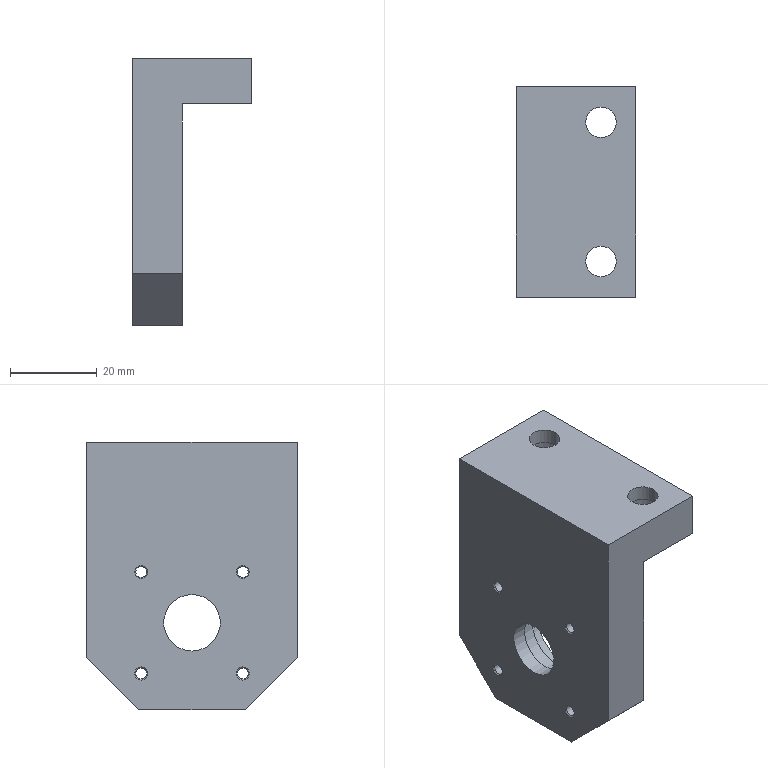Component | NX | CLHKJG_08_CYLINDER_SUPPORT | 1 solid | 33 faces | volume 36295 mm3 | plane 14 | cylinder 11 | cone 8 | commonest cylinder face diameters 2.5 x4 7 x2 10.5 x2 22 x1 13 x1 16 x1